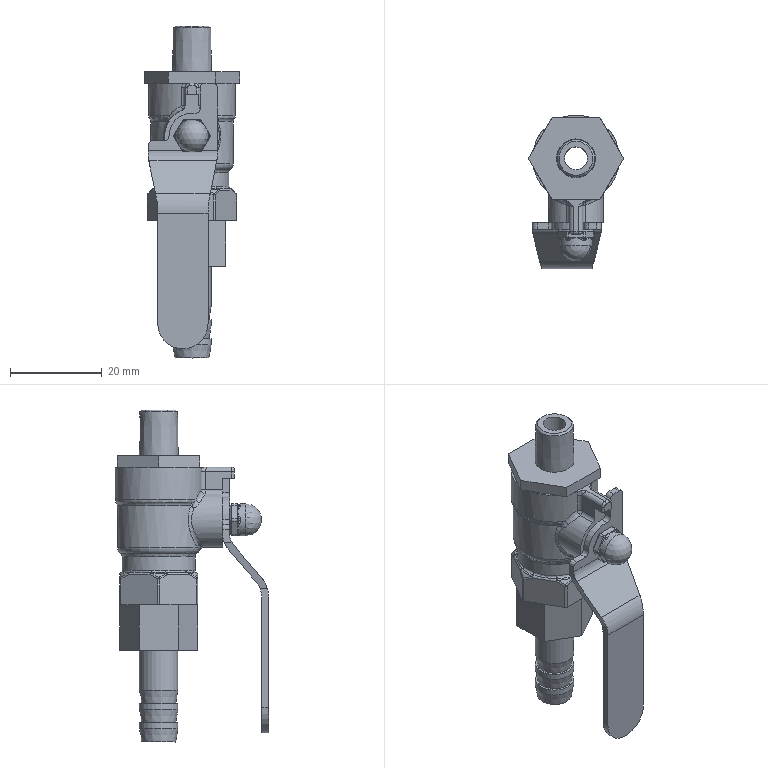Component | NX | VALVE | 3 solids | 254 faces | volume 11785 mm3 | plane 73 | spline 63 | cylinder 62 | sphere 23 | cone 17 | torus 16 | commonest cylinder face diameters 1 x20 0.6 x12 2 x11 10 x3 5 x3 8.4 x3 7 x2 11 x1